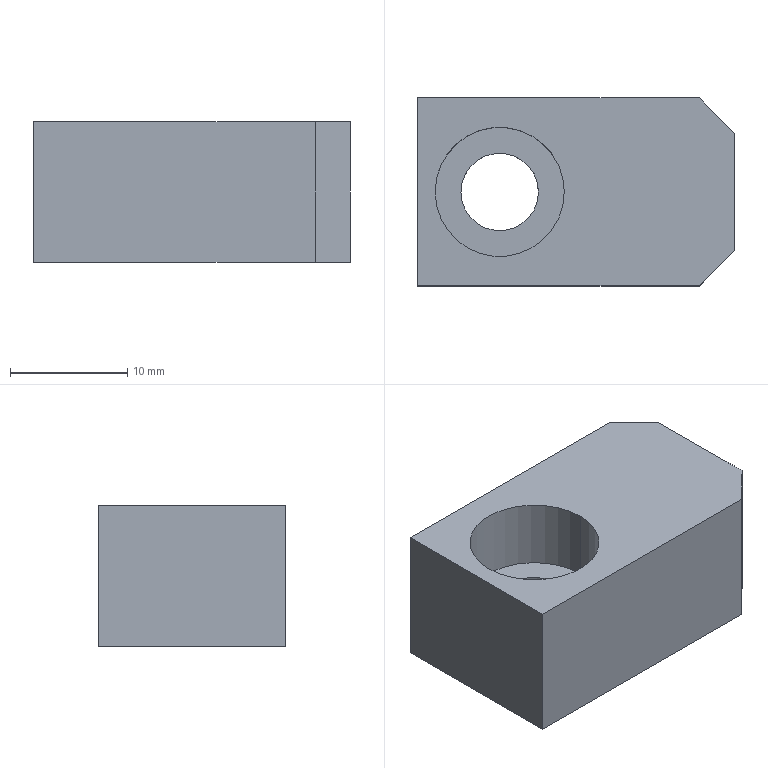Component | SolidWorks | STB-08-045-1 | 1 solid | 13 faces | box 27 x 16 x 12 mm | volume 4301 mm3 | plane 9 | cylinder 4 | commonest cylinder face diameters 11 x2 6.6 x2
build123d program:
from build123d import *

# Parameters (mm, degrees)
SKETCH1_W                                       = 27
SKETCH1_H                                       = 16
BOSS_EXTRUDE1_DEPTH                             = 6
M6_HEX_SOCKET_HEAD_CAP_SCREW_CBORE1_D           = 6.6
M6_HEX_SOCKET_HEAD_CAP_SCREW_CBORE1_CBORE_D     = 11
M6_HEX_SOCKET_HEAD_CAP_SCREW_CBORE1_CBORE_DEPTH = 6
CHAMFER1_SIZE                                   = 3


with BuildPart() as part:
    # Sketch1 → Boss-Extrude1 (new, symmetric)
    with BuildSketch(Plane(origin=(0, 0, 0), x_dir=(0, 0, -1), z_dir=(1, 0, 0))):
        Rectangle(SKETCH1_W, SKETCH1_H)
    extrude(amount=BOSS_EXTRUDE1_DEPTH, both=True)

    # M6 Hex Socket Head Cap Screw CBORE1 (through all)
    with Locations(Plane(origin=(6, 0, 0), x_dir=(0, 0, -1), z_dir=(1, 0, 0))):
        with Locations((-6.5, 0)):
            CounterBoreHole(M6_HEX_SOCKET_HEAD_CAP_SCREW_CBORE1_D / 2, M6_HEX_SOCKET_HEAD_CAP_SCREW_CBORE1_CBORE_D / 2, M6_HEX_SOCKET_HEAD_CAP_SCREW_CBORE1_CBORE_DEPTH)

    # Chamfer1
    chamfer1_edges = [part.edges().sort_by_distance(p)[0] for p in [
        (0, 8, -13.5),
        (0, -8, -13.5),
    ]]
    chamfer(chamfer1_edges, length=CHAMFER1_SIZE)


solid = part.part

# Placed as in the assembly
solid = solid.moved(Location((-241.404, 190.999, 24), (0, -90, 0)))
STEP:
#1=CARTESIAN_POINT('',(-9.977,7.52,0.9449));
#2=VERTEX_POINT('',#1);
#3=CARTESIAN_POINT('',(-9.543,7.52,0.9449));
#4=VERTEX_POINT('',#3);
#5=CARTESIAN_POINT('',(-9.76,7.52,0.9449));
#6=DIRECTION('',(0.,-0.,1.));
#7=DIRECTION('',(1.,0.,0.));
#8=AXIS2_PLACEMENT_3D('',#5,#6,#7);
#9=CIRCLE('',#8,0.2165);
#10=EDGE_CURVE('',#2,#4,#9,.T.);
#11=ORIENTED_EDGE('',*,*,#10,.F.);
#12=CARTESIAN_POINT('',(-9.977,7.52,1.181));
#13=VERTEX_POINT('',#12);
#14=CARTESIAN_POINT('',(-9.977,7.52,1.181));
#15=DIRECTION('',(0.,-0.,1.));
#16=VECTOR('',#15,39.37);
#17=LINE('',#14,#16);
#18=EDGE_CURVE('',#2,#13,#17,.T.);
#19=ORIENTED_EDGE('',*,*,#18,.T.);
#20=CARTESIAN_POINT('',(-9.543,7.52,1.181));
#21=VERTEX_POINT('',#20);
#22=CARTESIAN_POINT('',(-9.76,7.52,1.181));
#23=DIRECTION('',(0.,-0.,1.));
#24=DIRECTION('',(1.,0.,0.));
#25=AXIS2_PLACEMENT_3D('',#22,#23,#24);
#26=CIRCLE('',#25,0.2165);
#27=EDGE_CURVE('',#13,#21,#26,.T.);
#28=ORIENTED_EDGE('',*,*,#27,.T.);
#29=CARTESIAN_POINT('',(-9.543,7.52,1.181));
#30=DIRECTION('',(0.,-0.,1.));
#31=VECTOR('',#30,39.37);
#32=LINE('',#29,#31);
#33=EDGE_CURVE('',#4,#21,#32,.T.);
#34=ORIENTED_EDGE('',*,*,#33,.F.);
#35=EDGE_LOOP('',(#11,#19,#28,#34));
#36=FACE_OUTER_BOUND('',#35,.T.);
#37=CARTESIAN_POINT('',(-9.76,7.52,1.181));
#38=DIRECTION('',(0.,-0.,1.));
#39=DIRECTION('',(1.,0.,0.));
#40=AXIS2_PLACEMENT_3D('',#37,#38,#39);
#41=CYLINDRICAL_SURFACE('',#40,0.2165);
#42=ADVANCED_FACE('',(#36),#41,.F.);
#43=CARTESIAN_POINT('',(-9.89,7.52,0.7087));
#44=VERTEX_POINT('',#43);
#45=CARTESIAN_POINT('',(-9.63,7.52,0.7087));
#46=VERTEX_POINT('',#45);
#47=CARTESIAN_POINT('',(-9.76,7.52,0.7087));
#48=DIRECTION('',(0.,-0.,1.));
#49=DIRECTION('',(1.,0.,0.));
#50=AXIS2_PLACEMENT_3D('',#47,#48,#49);
#51=CIRCLE('',#50,0.1299);
#52=EDGE_CURVE('',#44,#46,#51,.T.);
#53=ORIENTED_EDGE('',*,*,#52,.F.);
#54=CARTESIAN_POINT('',(-9.89,7.52,0.9449));
#55=VERTEX_POINT('',#54);
#56=CARTESIAN_POINT('',(-9.89,7.52,1.181));
#57=DIRECTION('',(0.,-0.,1.));
#58=VECTOR('',#57,39.37);
#59=LINE('',#56,#58);
#60=EDGE_CURVE('',#44,#55,#59,.T.);
#61=ORIENTED_EDGE('',*,*,#60,.T.);
#62=CARTESIAN_POINT('',(-9.63,7.52,0.9449));
#63=VERTEX_POINT('',#62);
#64=CARTESIAN_POINT('',(-9.76,7.52,0.9449));
#65=DIRECTION('',(0.,-0.,1.));
#66=DIRECTION('',(1.,0.,0.));
#67=AXIS2_PLACEMENT_3D('',#64,#65,#66);
#68=CIRCLE('',#67,0.1299);
#69=EDGE_CURVE('',#55,#63,#68,.T.);
#70=ORIENTED_EDGE('',*,*,#69,.T.);
#71=CARTESIAN_POINT('',(-9.63,7.52,1.181));
#72=DIRECTION('',(0.,-0.,1.));
#73=VECTOR('',#72,39.37);
#74=LINE('',#71,#73);
#75=EDGE_CURVE('',#46,#63,#74,.T.);
#76=ORIENTED_EDGE('',*,*,#75,.F.);
#77=EDGE_LOOP('',(#53,#61,#70,#76));
#78=FACE_OUTER_BOUND('',#77,.T.);
#79=CARTESIAN_POINT('',(-9.76,7.52,1.181));
#80=DIRECTION('',(0.,-0.,1.));
#81=DIRECTION('',(1.,0.,0.));
#82=AXIS2_PLACEMENT_3D('',#79,#80,#81);
#83=CYLINDRICAL_SURFACE('',#82,0.1299);
#84=ADVANCED_FACE('',(#78),#83,.F.);
#85=CARTESIAN_POINT('',(-10.036,7.835,0.7087));
#86=VERTEX_POINT('',#85);
#87=CARTESIAN_POINT('',(-10.036,7.205,0.7087));
#88=VERTEX_POINT('',#87);
#89=CARTESIAN_POINT('',(-10.036,7.835,0.7087));
#90=DIRECTION('',(-0.,-1.,0.));
#91=VECTOR('',#90,39.37);
#92=LINE('',#89,#91);
#93=EDGE_CURVE('',#86,#88,#92,.T.);
#94=ORIENTED_EDGE('',*,*,#93,.T.);
#95=CARTESIAN_POINT('',(-10.036,7.205,1.181));
#96=VERTEX_POINT('',#95);
#97=CARTESIAN_POINT('',(-10.036,7.205,1.181));
#98=DIRECTION('',(-0.,0.,-1.));
#99=VECTOR('',#98,39.37);
#100=LINE('',#97,#99);
#101=EDGE_CURVE('',#96,#88,#100,.T.);
#102=ORIENTED_EDGE('',*,*,#101,.F.);
#103=CARTESIAN_POINT('',(-10.036,7.835,1.181));
#104=VERTEX_POINT('',#103);
#105=CARTESIAN_POINT('',(-10.036,7.835,1.181));
#106=DIRECTION('',(-0.,-1.,0.));
#107=VECTOR('',#106,39.37);
#108=LINE('',#105,#107);
#109=EDGE_CURVE('',#104,#96,#108,.T.);
#110=ORIENTED_EDGE('',*,*,#109,.F.);
#111=CARTESIAN_POINT('',(-10.036,7.835,1.181));
#112=DIRECTION('',(-0.,0.,-1.));
#113=VECTOR('',#112,39.37);
#114=LINE('',#111,#113);
#115=EDGE_CURVE('',#104,#86,#114,.T.);
#116=ORIENTED_EDGE('',*,*,#115,.T.);
#117=EDGE_LOOP('',(#94,#102,#110,#116));
#118=FACE_OUTER_BOUND('',#117,.T.);
#119=CARTESIAN_POINT('',(-10.036,7.835,1.181));
#120=DIRECTION('',(1.,-0.,-0.));
#121=DIRECTION('',(-0.,0.,-1.));
#122=AXIS2_PLACEMENT_3D('',#119,#120,#121);
#123=PLANE('',#122);
#124=ADVANCED_FACE('',(#118),#123,.F.);
#125=CARTESIAN_POINT('',(-9.091,7.205,0.7087));
#126=VERTEX_POINT('',#125);
#127=CARTESIAN_POINT('',(-10.036,7.205,0.7087));
#128=DIRECTION('',(1.,-0.,-0.));
#129=VECTOR('',#128,39.37);
#130=LINE('',#127,#129);
#131=EDGE_CURVE('',#88,#126,#130,.T.);
#132=ORIENTED_EDGE('',*,*,#131,.T.);
#133=CARTESIAN_POINT('',(-9.091,7.205,1.181));
#134=VERTEX_POINT('',#133);
#135=CARTESIAN_POINT('',(-9.091,7.205,1.181));
#136=DIRECTION('',(0.,-0.,1.));
#137=VECTOR('',#136,39.37);
#138=LINE('',#135,#137);
#139=EDGE_CURVE('',#126,#134,#138,.T.);
#140=ORIENTED_EDGE('',*,*,#139,.T.);
#141=CARTESIAN_POINT('',(-10.036,7.205,1.181));
#142=DIRECTION('',(1.,-0.,-0.));
#143=VECTOR('',#142,39.37);
#144=LINE('',#141,#143);
#145=EDGE_CURVE('',#96,#134,#144,.T.);
#146=ORIENTED_EDGE('',*,*,#145,.F.);
#147=ORIENTED_EDGE('',*,*,#101,.T.);
#148=EDGE_LOOP('',(#132,#140,#146,#147));
#149=FACE_OUTER_BOUND('',#148,.T.);
#150=CARTESIAN_POINT('',(-10.036,7.205,1.181));
#151=DIRECTION('',(0.,1.,-0.));
#152=DIRECTION('',(-1.,0.,0.));
#153=AXIS2_PLACEMENT_3D('',#150,#151,#152);
#154=PLANE('',#153);
#155=ADVANCED_FACE('',(#149),#154,.F.);
#156=CARTESIAN_POINT('',(-8.973,7.323,1.181));
#157=VERTEX_POINT('',#156);
#158=CARTESIAN_POINT('',(-8.973,7.716,1.181));
#159=VERTEX_POINT('',#158);
#160=CARTESIAN_POINT('',(-8.973,7.835,1.181));
#161=DIRECTION('',(-0.,1.,-0.));
#162=VECTOR('',#161,39.37);
#163=LINE('',#160,#162);
#164=EDGE_CURVE('',#157,#159,#163,.T.);
#165=ORIENTED_EDGE('',*,*,#164,.F.);
#166=CARTESIAN_POINT('',(-8.973,7.323,0.7087));
#167=VERTEX_POINT('',#166);
#168=CARTESIAN_POINT('',(-8.973,7.323,1.181));
#169=DIRECTION('',(-0.,0.,-1.));
#170=VECTOR('',#169,39.37);
#171=LINE('',#168,#170);
#172=EDGE_CURVE('',#157,#167,#171,.T.);
#173=ORIENTED_EDGE('',*,*,#172,.T.);
#174=CARTESIAN_POINT('',(-8.973,7.716,0.7087));
#175=VERTEX_POINT('',#174);
#176=CARTESIAN_POINT('',(-8.973,7.835,0.7087));
#177=DIRECTION('',(-0.,1.,-0.));
#178=VECTOR('',#177,39.37);
#179=LINE('',#176,#178);
#180=EDGE_CURVE('',#167,#175,#179,.T.);
#181=ORIENTED_EDGE('',*,*,#180,.T.);
#182=CARTESIAN_POINT('',(-8.973,7.716,1.181));
#183=DIRECTION('',(0.,-0.,1.));
#184=VECTOR('',#183,39.37);
#185=LINE('',#182,#184);
#186=EDGE_CURVE('',#175,#159,#185,.T.);
#187=ORIENTED_EDGE('',*,*,#186,.T.);
#188=EDGE_LOOP('',(#165,#173,#181,#187));
#189=FACE_OUTER_BOUND('',#188,.T.);
#190=CARTESIAN_POINT('',(-8.973,7.835,1.181));
#191=DIRECTION('',(-1.,-0.,0.));
#192=DIRECTION('',(0.,-1.,0.));
#193=AXIS2_PLACEMENT_3D('',#190,#191,#192);
#194=PLANE('',#193);
#195=ADVANCED_FACE('',(#189),#194,.F.);
#196=CARTESIAN_POINT('',(-9.091,7.835,1.181));
#197=VERTEX_POINT('',#196);
#198=CARTESIAN_POINT('',(-10.036,7.835,1.181));
#199=DIRECTION('',(-1.,0.,0.));
#200=VECTOR('',#199,39.37);
#201=LINE('',#198,#200);
#202=EDGE_CURVE('',#197,#104,#201,.T.);
#203=ORIENTED_EDGE('',*,*,#202,.F.);
#204=CARTESIAN_POINT('',(-9.091,7.835,0.7087));
#205=VERTEX_POINT('',#204);
#206=CARTESIAN_POINT('',(-9.091,7.835,1.181));
#207=DIRECTION('',(-0.,0.,-1.));
#208=VECTOR('',#207,39.37);
#209=LINE('',#206,#208);
#210=EDGE_CURVE('',#197,#205,#209,.T.);
#211=ORIENTED_EDGE('',*,*,#210,.T.);
#212=CARTESIAN_POINT('',(-10.036,7.835,0.7087));
#213=DIRECTION('',(-1.,0.,0.));
#214=VECTOR('',#213,39.37);
#215=LINE('',#212,#214);
#216=EDGE_CURVE('',#205,#86,#215,.T.);
#217=ORIENTED_EDGE('',*,*,#216,.T.);
#218=ORIENTED_EDGE('',*,*,#115,.F.);
#219=EDGE_LOOP('',(#203,#211,#217,#218));
#220=FACE_OUTER_BOUND('',#219,.T.);
#221=CARTESIAN_POINT('',(-10.036,7.835,1.181));
#222=DIRECTION('',(-0.,-1.,0.));
#223=DIRECTION('',(1.,-0.,-0.));
#224=AXIS2_PLACEMENT_3D('',#221,#222,#223);
#225=PLANE('',#224);
#226=ADVANCED_FACE('',(#220),#225,.F.);
#227=CARTESIAN_POINT('',(-9.76,7.52,1.181));
#228=DIRECTION('',(0.,-0.,1.));
#229=DIRECTION('',(1.,0.,0.));
#230=AXIS2_PLACEMENT_3D('',#227,#228,#229);
#231=CIRCLE('',#230,0.2165);
#232=EDGE_CURVE('',#21,#13,#231,.T.);
#233=ORIENTED_EDGE('',*,*,#232,.F.);
#234=ORIENTED_EDGE('',*,*,#27,.F.);
#235=EDGE_LOOP('',(#233,#234));
#236=FACE_BOUND('',#235,.T.);
#237=ORIENTED_EDGE('',*,*,#145,.T.);
#238=CARTESIAN_POINT('',(-9.563,6.732,1.181));
#239=DIRECTION('',(0.7071,0.7071,-0.));
#240=VECTOR('',#239,39.37);
#241=LINE('',#238,#240);
#242=EDGE_CURVE('',#134,#157,#241,.T.);
#243=ORIENTED_EDGE('',*,*,#242,.T.);
#244=ORIENTED_EDGE('',*,*,#164,.T.);
#245=CARTESIAN_POINT('',(-9.248,7.992,1.181));
#246=DIRECTION('',(-0.7071,0.7071,0.));
#247=VECTOR('',#246,39.37);
#248=LINE('',#245,#247);
#249=EDGE_CURVE('',#159,#197,#248,.T.);
#250=ORIENTED_EDGE('',*,*,#249,.T.);
#251=ORIENTED_EDGE('',*,*,#202,.T.);
#252=ORIENTED_EDGE('',*,*,#109,.T.);
#253=EDGE_LOOP('',(#237,#243,#244,#250,#251,#252));
#254=FACE_OUTER_BOUND('',#253,.T.);
#255=CARTESIAN_POINT('',(-10.036,7.205,1.181));
#256=DIRECTION('',(0.,-0.,1.));
#257=DIRECTION('',(1.,-0.,-0.));
#258=AXIS2_PLACEMENT_3D('',#255,#256,#257);
#259=PLANE('',#258);
#260=ADVANCED_FACE('',(#236,#254),#259,.T.);
#261=CARTESIAN_POINT('',(-9.76,7.52,0.7087));
#262=DIRECTION('',(0.,-0.,1.));
#263=DIRECTION('',(1.,0.,0.));
#264=AXIS2_PLACEMENT_3D('',#261,#262,#263);
#265=CIRCLE('',#264,0.1299);
#266=EDGE_CURVE('',#46,#44,#265,.T.);
#267=ORIENTED_EDGE('',*,*,#266,.T.);
#268=ORIENTED_EDGE('',*,*,#52,.T.);
#269=EDGE_LOOP('',(#267,#268));
#270=FACE_BOUND('',#269,.T.);
#271=ORIENTED_EDGE('',*,*,#180,.F.);
#272=CARTESIAN_POINT('',(-8.973,7.323,0.7087));
#273=DIRECTION('',(-0.7071,-0.7071,0.));
#274=VECTOR('',#273,39.37);
#275=LINE('',#272,#274);
#276=EDGE_CURVE('',#167,#126,#275,.T.);
#277=ORIENTED_EDGE('',*,*,#276,.T.);
#278=ORIENTED_EDGE('',*,*,#131,.F.);
#279=ORIENTED_EDGE('',*,*,#93,.F.);
#280=ORIENTED_EDGE('',*,*,#216,.F.);
#281=CARTESIAN_POINT('',(-9.091,7.835,0.7087));
#282=DIRECTION('',(0.7071,-0.7071,-0.));
#283=VECTOR('',#282,39.37);
#284=LINE('',#281,#283);
#285=EDGE_CURVE('',#205,#175,#284,.T.);
#286=ORIENTED_EDGE('',*,*,#285,.T.);
#287=EDGE_LOOP('',(#271,#277,#278,#279,#280,#286));
#288=FACE_OUTER_BOUND('',#287,.T.);
#289=CARTESIAN_POINT('',(-10.036,7.205,0.7087));
#290=DIRECTION('',(0.,-0.,1.));
#291=DIRECTION('',(1.,-0.,-0.));
#292=AXIS2_PLACEMENT_3D('',#289,#290,#291);
#293=PLANE('',#292);
#294=ADVANCED_FACE('',(#270,#288),#293,.F.);
#295=ORIENTED_EDGE('',*,*,#60,.F.);
#296=ORIENTED_EDGE('',*,*,#266,.F.);
#297=ORIENTED_EDGE('',*,*,#75,.T.);
#298=CARTESIAN_POINT('',(-9.76,7.52,0.9449));
#299=DIRECTION('',(0.,-0.,1.));
#300=DIRECTION('',(1.,0.,0.));
#301=AXIS2_PLACEMENT_3D('',#298,#299,#300);
#302=CIRCLE('',#301,0.1299);
#303=EDGE_CURVE('',#63,#55,#302,.T.);
#304=ORIENTED_EDGE('',*,*,#303,.T.);
#305=EDGE_LOOP('',(#295,#296,#297,#304));
#306=FACE_OUTER_BOUND('',#305,.T.);
#307=CARTESIAN_POINT('',(-9.76,7.52,1.181));
#308=DIRECTION('',(0.,-0.,1.));
#309=DIRECTION('',(1.,0.,0.));
#310=AXIS2_PLACEMENT_3D('',#307,#308,#309);
#311=CYLINDRICAL_SURFACE('',#310,0.1299);
#312=ADVANCED_FACE('',(#306),#311,.F.);
#313=ORIENTED_EDGE('',*,*,#303,.F.);
#314=ORIENTED_EDGE('',*,*,#69,.F.);
#315=EDGE_LOOP('',(#313,#314));
#316=FACE_BOUND('',#315,.T.);
#317=CARTESIAN_POINT('',(-9.76,7.52,0.9449));
#318=DIRECTION('',(0.,-0.,1.));
#319=DIRECTION('',(1.,0.,0.));
#320=AXIS2_PLACEMENT_3D('',#317,#318,#319);
#321=CIRCLE('',#320,0.2165);
#322=EDGE_CURVE('',#4,#2,#321,.T.);
#323=ORIENTED_EDGE('',*,*,#322,.T.);
#324=ORIENTED_EDGE('',*,*,#10,.T.);
#325=EDGE_LOOP('',(#323,#324));
#326=FACE_OUTER_BOUND('',#325,.T.);
#327=CARTESIAN_POINT('',(-9.76,7.65,0.9449));
#328=DIRECTION('',(-0.,0.,-1.));
#329=DIRECTION('',(-1.,0.,0.));
#330=AXIS2_PLACEMENT_3D('',#327,#328,#329);
#331=PLANE('',#330);
#332=ADVANCED_FACE('',(#316,#326),#331,.F.);
#333=ORIENTED_EDGE('',*,*,#18,.F.);
#334=ORIENTED_EDGE('',*,*,#322,.F.);
#335=ORIENTED_EDGE('',*,*,#33,.T.);
#336=ORIENTED_EDGE('',*,*,#232,.T.);
#337=EDGE_LOOP('',(#333,#334,#335,#336));
#338=FACE_OUTER_BOUND('',#337,.T.);
#339=CARTESIAN_POINT('',(-9.76,7.52,1.181));
#340=DIRECTION('',(0.,-0.,1.));
#341=DIRECTION('',(1.,0.,0.));
#342=AXIS2_PLACEMENT_3D('',#339,#340,#341);
#343=CYLINDRICAL_SURFACE('',#342,0.2165);
#344=ADVANCED_FACE('',(#338),#343,.F.);
#345=ORIENTED_EDGE('',*,*,#242,.F.);
#346=ORIENTED_EDGE('',*,*,#139,.F.);
#347=ORIENTED_EDGE('',*,*,#276,.F.);
#348=ORIENTED_EDGE('',*,*,#172,.F.);
#349=EDGE_LOOP('',(#345,#346,#347,#348));
#350=FACE_OUTER_BOUND('',#349,.T.);
#351=CARTESIAN_POINT('',(-8.973,7.323,1.181));
#352=DIRECTION('',(-0.7071,0.7071,0.));
#353=DIRECTION('',(-0.7071,-0.7071,0.));
#354=AXIS2_PLACEMENT_3D('',#351,#352,#353);
#355=PLANE('',#354);
#356=ADVANCED_FACE('',(#350),#355,.F.);
#357=ORIENTED_EDGE('',*,*,#249,.F.);
#358=ORIENTED_EDGE('',*,*,#186,.F.);
#359=ORIENTED_EDGE('',*,*,#285,.F.);
#360=ORIENTED_EDGE('',*,*,#210,.F.);
#361=EDGE_LOOP('',(#357,#358,#359,#360));
#362=FACE_OUTER_BOUND('',#361,.T.);
#363=CARTESIAN_POINT('',(-9.091,7.835,1.181));
#364=DIRECTION('',(-0.7071,-0.7071,0.));
#365=DIRECTION('',(0.7071,-0.7071,-0.));
#366=AXIS2_PLACEMENT_3D('',#363,#364,#365);
#367=PLANE('',#366);
#368=ADVANCED_FACE('',(#362),#367,.F.);
#369=CLOSED_SHELL('',(#42,#84,#124,#155,#195,#226,#260,#294,#312,#332,#344,#356,#368));
#370=MANIFOLD_SOLID_BREP('',#369);
#371=CARTESIAN_POINT('',(0.,0.,0.));
#372=DIRECTION('',(0.,0.,1.));
#373=DIRECTION('',(1.,0.,0.));
#374=AXIS2_PLACEMENT_3D('',#371,#372,#373);
#375=(LENGTH_UNIT()NAMED_UNIT(*)SI_UNIT($,.METRE.));
#376=LENGTH_MEASURE_WITH_UNIT(LENGTH_MEASURE(0.0254),#375);
#377=DIMENSIONAL_EXPONENTS(1.,0.,0.,0.,0.,0.,0.);
#378=(CONVERSION_BASED_UNIT('',#376)LENGTH_UNIT()NAMED_UNIT(#377));
#379=UNCERTAINTY_MEASURE_WITH_UNIT(LENGTH_MEASURE(0.00001),#378,'','');
#380=(NAMED_UNIT(*)PLANE_ANGLE_UNIT()SI_UNIT($,.RADIAN.));
#381=(NAMED_UNIT(*)SI_UNIT($,.STERADIAN.)SOLID_ANGLE_UNIT());
#382=(GEOMETRIC_REPRESENTATION_CONTEXT(3)GLOBAL_UNCERTAINTY_ASSIGNED_CONTEXT((#379))GLOBAL_UNIT_ASSIGNED_CONTEXT((#378,#380,#381))REPRESENTATION_CONTEXT('',''));
#383=ADVANCED_BREP_SHAPE_REPRESENTATION('',(#370,#374),#382);
#384=COLOUR_RGB('',0.7922,0.8196,0.9333);
#385=FILL_AREA_STYLE_COLOUR('',#384);
#386=FILL_AREA_STYLE('',(#385));
#387=SURFACE_STYLE_FILL_AREA(#386);
#388=SURFACE_SIDE_STYLE('',(#387));
#389=SURFACE_STYLE_USAGE(.BOTH.,#388);
#390=PRESENTATION_STYLE_ASSIGNMENT((#389));
#391=STYLED_ITEM('',(#390),#370);
#392=(LENGTH_UNIT()NAMED_UNIT(*)SI_UNIT($,.METRE.));
#393=LENGTH_MEASURE_WITH_UNIT(LENGTH_MEASURE(0.0254),#392);
#394=DIMENSIONAL_EXPONENTS(1.,0.,0.,0.,0.,0.,0.);
#395=(CONVERSION_BASED_UNIT('',#393)LENGTH_UNIT()NAMED_UNIT(#394));
#396=UNCERTAINTY_MEASURE_WITH_UNIT(LENGTH_MEASURE(0.00001),#395,'','');
#397=(NAMED_UNIT(*)PLANE_ANGLE_UNIT()SI_UNIT($,.RADIAN.));
#398=(NAMED_UNIT(*)SI_UNIT($,.STERADIAN.)SOLID_ANGLE_UNIT());
#399=(GEOMETRIC_REPRESENTATION_CONTEXT(3)GLOBAL_UNCERTAINTY_ASSIGNED_CONTEXT((#396))GLOBAL_UNIT_ASSIGNED_CONTEXT((#395,#397,#398))REPRESENTATION_CONTEXT('',''));
#400=MECHANICAL_DESIGN_GEOMETRIC_PRESENTATION_REPRESENTATION('',(#391),#399);
#401=PRESENTATION_LAYER_ASSIGNMENT('','',(#391));